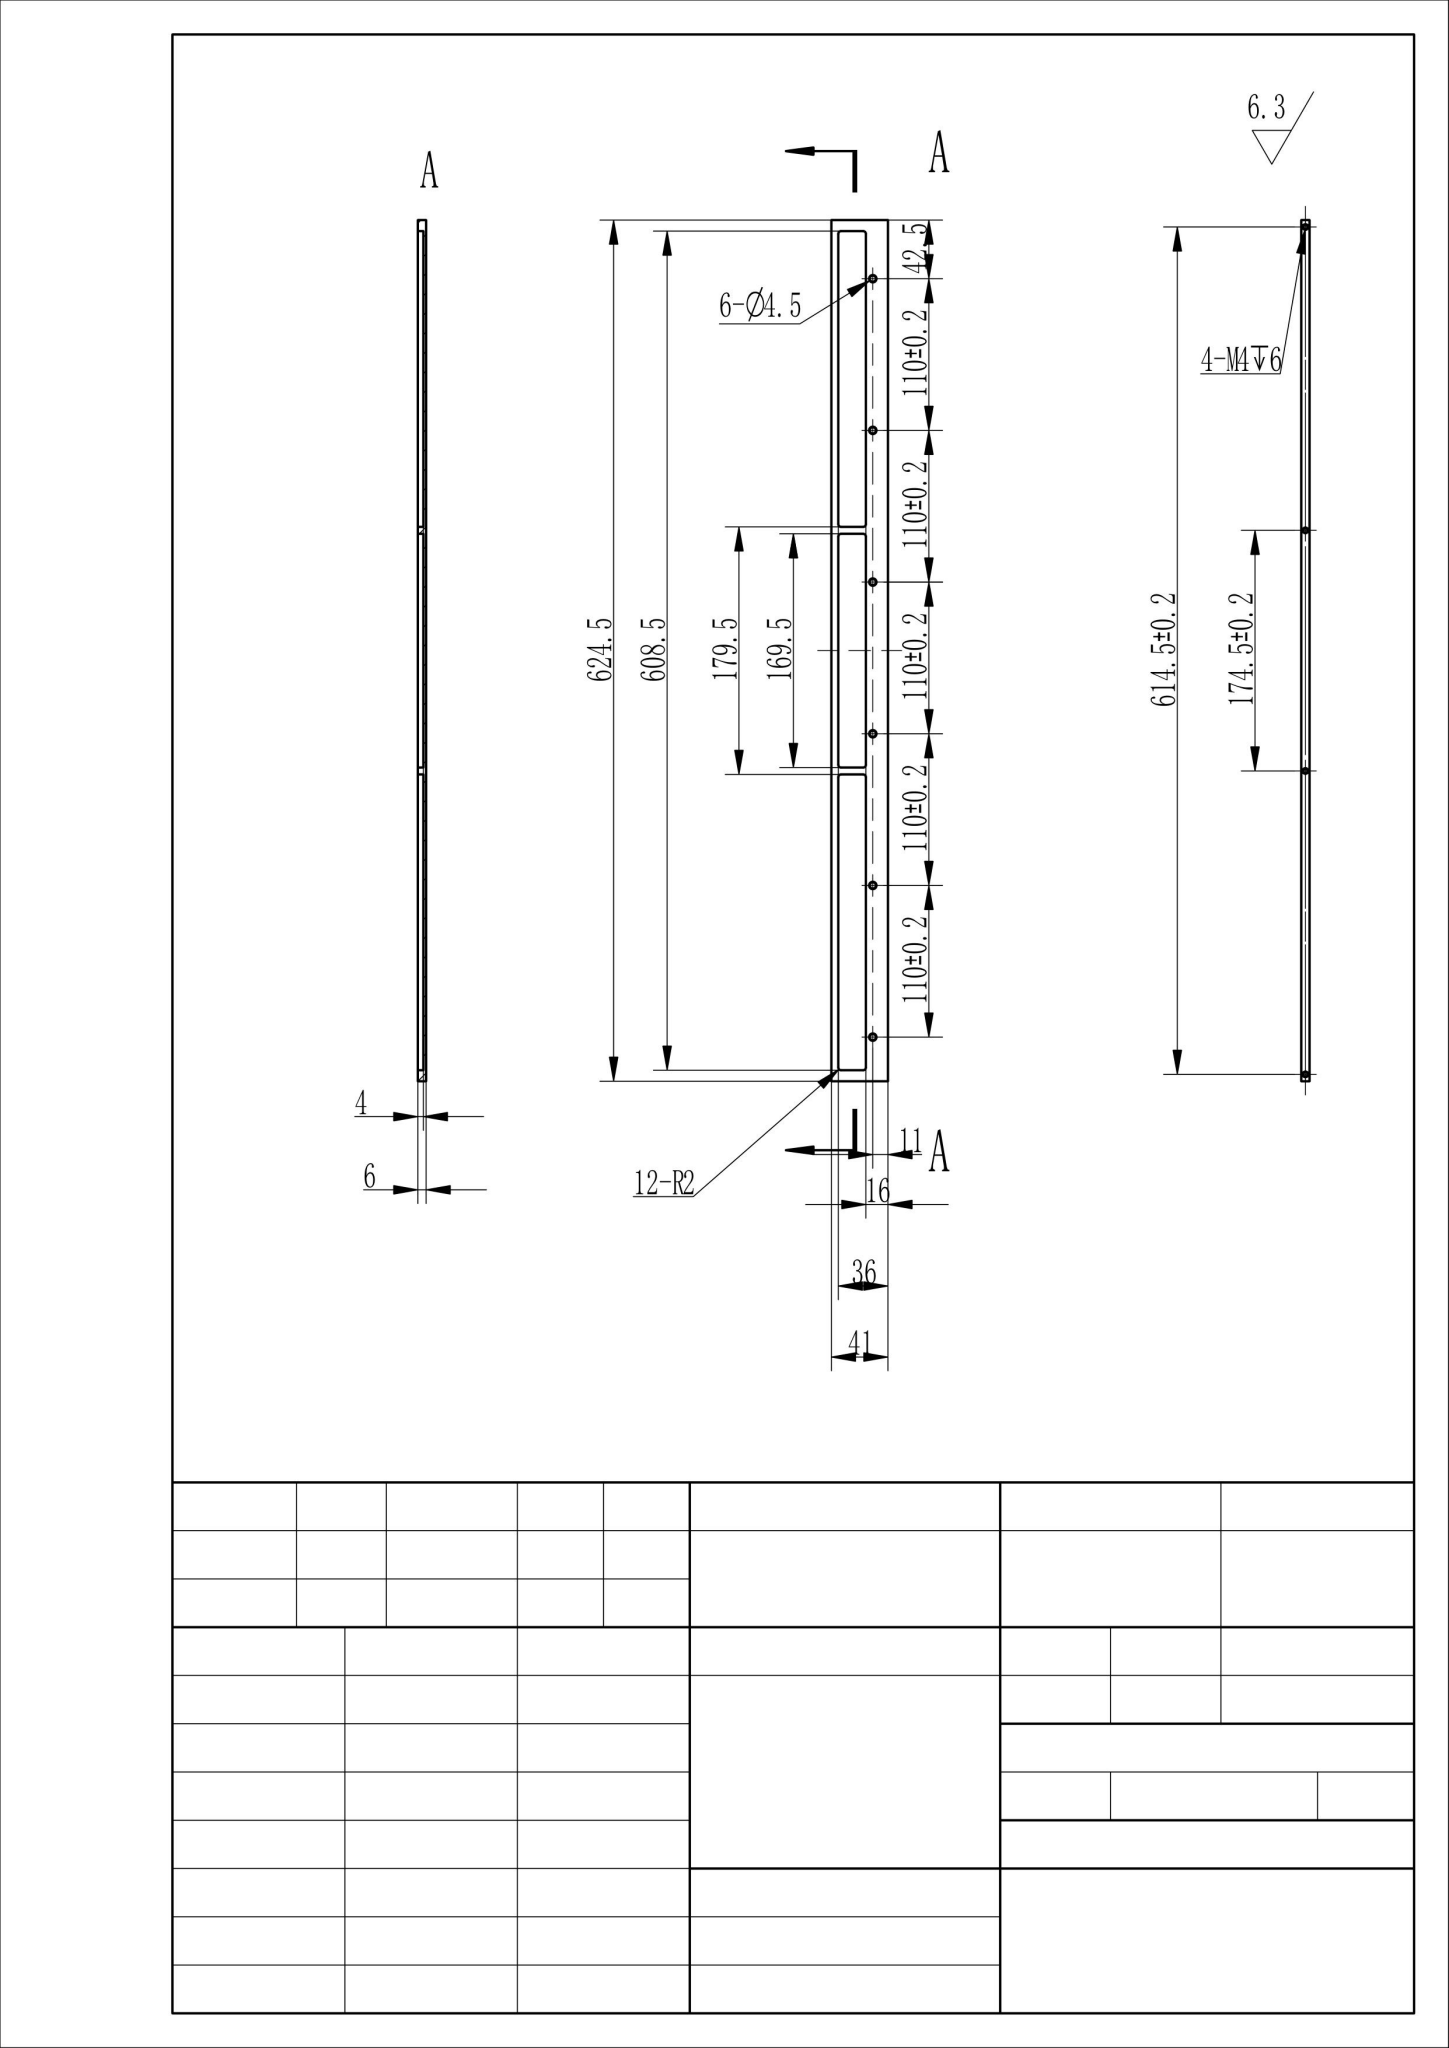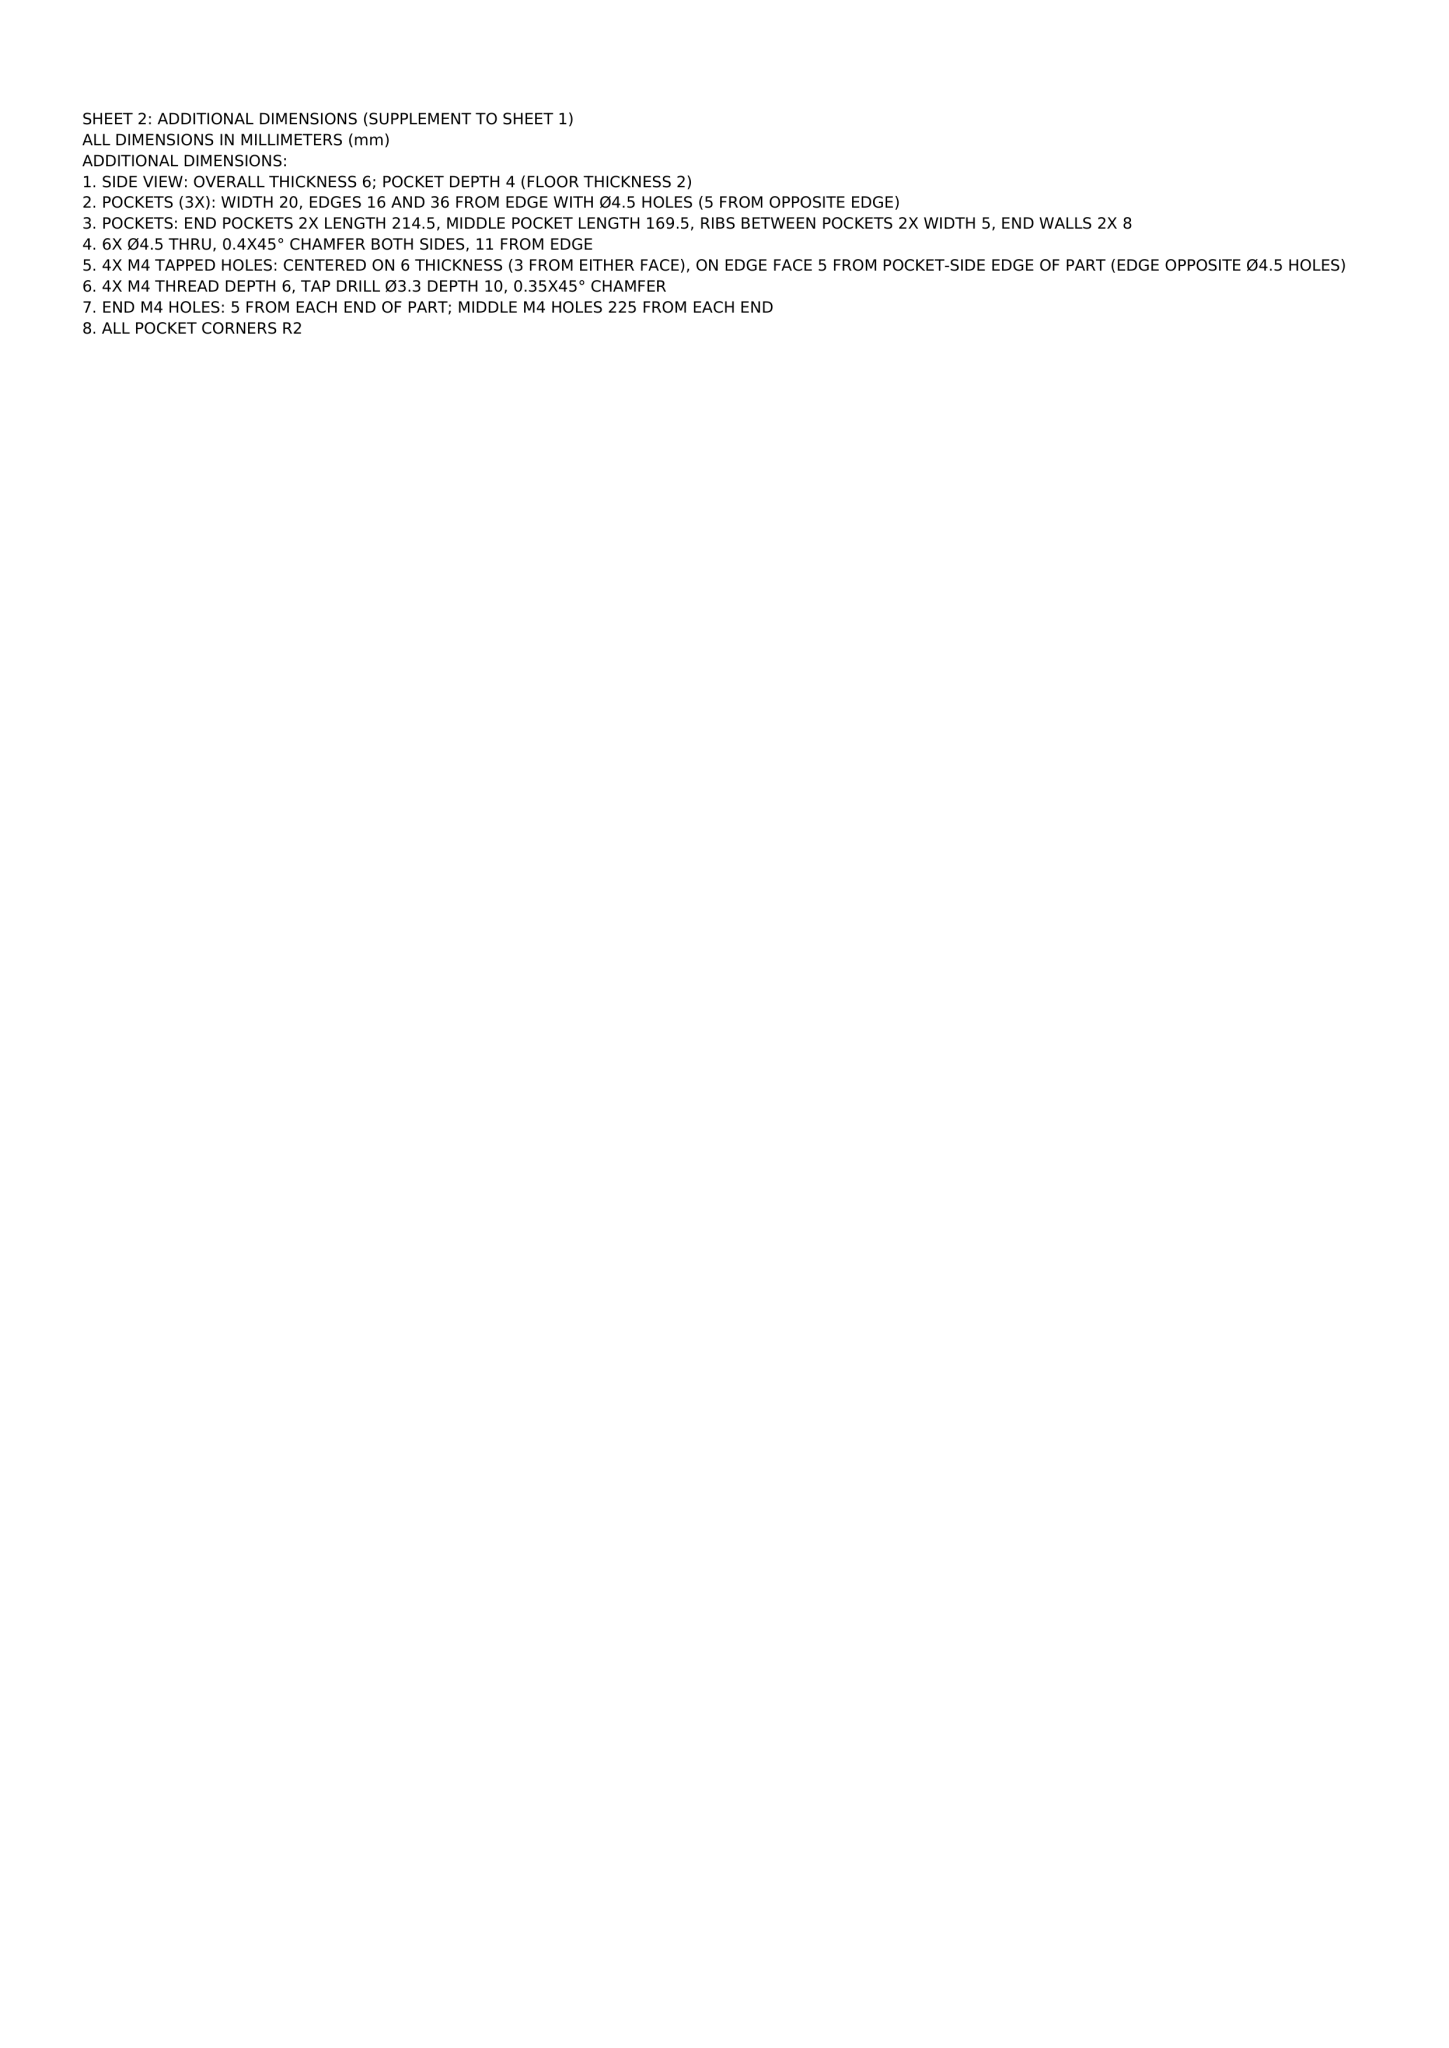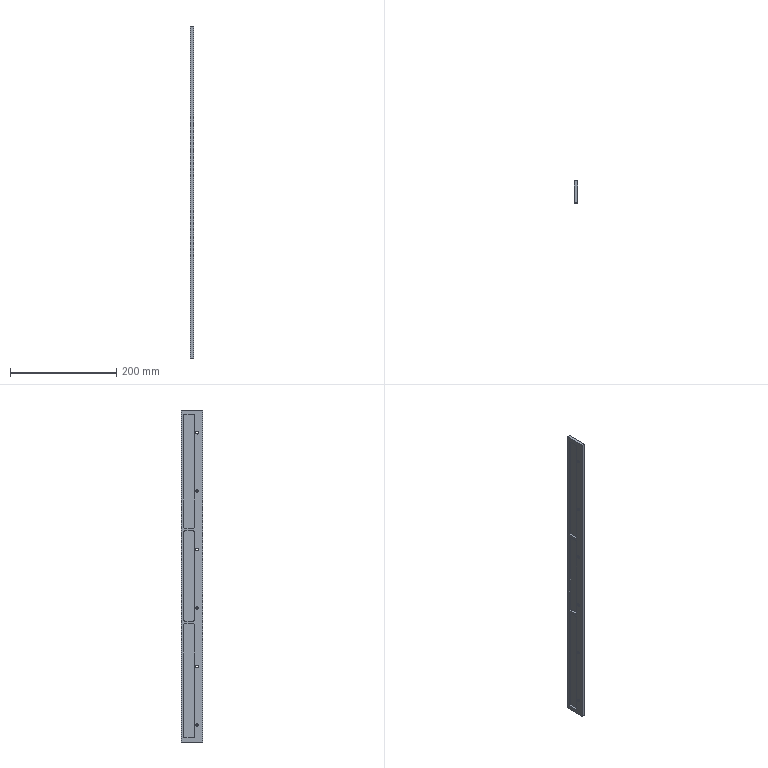Part | NX | mm | 1 solid | 63 faces | box 6 x 41 x 624.5 mm | volume 104845 mm3 | cylinder 22 | plane 21 | cone 20 | commonest cylinder face diameters 4 x12 4.5 x6 3.3 x4